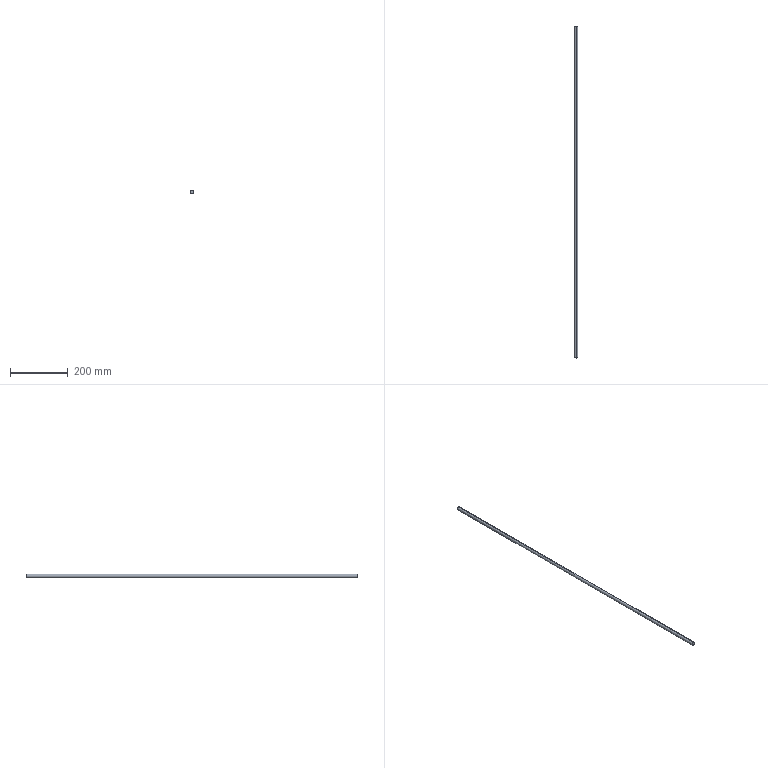Component | SolidWorks | JL001-05-01-002-1 | 1 solid | 4 faces | box 12 x 1150 x 12 mm | volume 130062 mm3 | cylinder 2 | plane 2 | commonest cylinder face diameters 12 x2
build123d program:
from build123d import *

# Parameters (mm, degrees)
SKETCH1_R           = 6
BOSS_EXTRUDE1_DEPTH = 1150


with BuildPart() as part:
    # Sketch1 → Boss-Extrude1 (new body)
    with BuildSketch(Plane(origin=(0, 0, 0), x_dir=(1, 0, 0), z_dir=(0, 1, 0))):
        with Locations(Location((0, 0, 0), (0, 0, 270))):
            Circle(SKETCH1_R)
    extrude(amount=BOSS_EXTRUDE1_DEPTH)


solid = part.part

# Placed as in the assembly
solid = solid.moved(Location((0, -10, 105), (0, 0, 0)))
STEP:
#1=CARTESIAN_POINT('',(0.,44.882,4.37));
#2=VERTEX_POINT('',#1);
#3=CARTESIAN_POINT('',(0.,44.882,3.898));
#4=VERTEX_POINT('',#3);
#5=CARTESIAN_POINT('',(0.,44.882,4.134));
#6=DIRECTION('',(0.,1.,0.));
#7=DIRECTION('',(0.,0.,1.));
#8=AXIS2_PLACEMENT_3D('',#5,#6,#7);
#9=CIRCLE('',#8,0.2362);
#10=EDGE_CURVE('',#2,#4,#9,.T.);
#11=ORIENTED_EDGE('',*,*,#10,.F.);
#12=CARTESIAN_POINT('',(0.,-0.3937,4.37));
#13=VERTEX_POINT('',#12);
#14=CARTESIAN_POINT('',(0.,44.882,4.37));
#15=DIRECTION('',(0.,-1.,0.));
#16=VECTOR('',#15,39.37);
#17=LINE('',#14,#16);
#18=EDGE_CURVE('',#2,#13,#17,.T.);
#19=ORIENTED_EDGE('',*,*,#18,.T.);
#20=CARTESIAN_POINT('',(0.,-0.3937,3.898));
#21=VERTEX_POINT('',#20);
#22=CARTESIAN_POINT('',(0.,-0.3937,4.134));
#23=DIRECTION('',(0.,1.,0.));
#24=DIRECTION('',(0.,0.,1.));
#25=AXIS2_PLACEMENT_3D('',#22,#23,#24);
#26=CIRCLE('',#25,0.2362);
#27=EDGE_CURVE('',#13,#21,#26,.T.);
#28=ORIENTED_EDGE('',*,*,#27,.T.);
#29=CARTESIAN_POINT('',(0.,44.882,3.898));
#30=DIRECTION('',(0.,-1.,0.));
#31=VECTOR('',#30,39.37);
#32=LINE('',#29,#31);
#33=EDGE_CURVE('',#4,#21,#32,.T.);
#34=ORIENTED_EDGE('',*,*,#33,.F.);
#35=EDGE_LOOP('',(#11,#19,#28,#34));
#36=FACE_OUTER_BOUND('',#35,.T.);
#37=CARTESIAN_POINT('',(0.,44.882,4.134));
#38=DIRECTION('',(0.,-1.,0.));
#39=DIRECTION('',(0.,0.,-1.));
#40=AXIS2_PLACEMENT_3D('',#37,#38,#39);
#41=CYLINDRICAL_SURFACE('',#40,0.2362);
#42=ADVANCED_FACE('',(#36),#41,.T.);
#43=ORIENTED_EDGE('',*,*,#18,.F.);
#44=CARTESIAN_POINT('',(0.,44.882,4.134));
#45=DIRECTION('',(0.,1.,0.));
#46=DIRECTION('',(0.,0.,1.));
#47=AXIS2_PLACEMENT_3D('',#44,#45,#46);
#48=CIRCLE('',#47,0.2362);
#49=EDGE_CURVE('',#4,#2,#48,.T.);
#50=ORIENTED_EDGE('',*,*,#49,.F.);
#51=ORIENTED_EDGE('',*,*,#33,.T.);
#52=CARTESIAN_POINT('',(0.,-0.3937,4.134));
#53=DIRECTION('',(0.,1.,0.));
#54=DIRECTION('',(0.,0.,1.));
#55=AXIS2_PLACEMENT_3D('',#52,#53,#54);
#56=CIRCLE('',#55,0.2362);
#57=EDGE_CURVE('',#21,#13,#56,.T.);
#58=ORIENTED_EDGE('',*,*,#57,.T.);
#59=EDGE_LOOP('',(#43,#50,#51,#58));
#60=FACE_OUTER_BOUND('',#59,.T.);
#61=CARTESIAN_POINT('',(0.,44.882,4.134));
#62=DIRECTION('',(0.,-1.,0.));
#63=DIRECTION('',(0.,0.,-1.));
#64=AXIS2_PLACEMENT_3D('',#61,#62,#63);
#65=CYLINDRICAL_SURFACE('',#64,0.2362);
#66=ADVANCED_FACE('',(#60),#65,.T.);
#67=ORIENTED_EDGE('',*,*,#49,.T.);
#68=ORIENTED_EDGE('',*,*,#10,.T.);
#69=EDGE_LOOP('',(#67,#68));
#70=FACE_OUTER_BOUND('',#69,.T.);
#71=CARTESIAN_POINT('',(0.,44.882,4.134));
#72=DIRECTION('',(0.,1.,0.));
#73=DIRECTION('',(0.,0.,1.));
#74=AXIS2_PLACEMENT_3D('',#71,#72,#73);
#75=PLANE('',#74);
#76=ADVANCED_FACE('',(#70),#75,.T.);
#77=ORIENTED_EDGE('',*,*,#57,.F.);
#78=ORIENTED_EDGE('',*,*,#27,.F.);
#79=EDGE_LOOP('',(#77,#78));
#80=FACE_OUTER_BOUND('',#79,.T.);
#81=CARTESIAN_POINT('',(0.,-0.3937,4.134));
#82=DIRECTION('',(0.,1.,0.));
#83=DIRECTION('',(0.,0.,1.));
#84=AXIS2_PLACEMENT_3D('',#81,#82,#83);
#85=PLANE('',#84);
#86=ADVANCED_FACE('',(#80),#85,.F.);
#87=CLOSED_SHELL('',(#42,#66,#76,#86));
#88=MANIFOLD_SOLID_BREP('',#87);
#89=CARTESIAN_POINT('',(0.,0.,0.));
#90=DIRECTION('',(0.,0.,1.));
#91=DIRECTION('',(1.,0.,0.));
#92=AXIS2_PLACEMENT_3D('',#89,#90,#91);
#93=(LENGTH_UNIT()NAMED_UNIT(*)SI_UNIT($,.METRE.));
#94=LENGTH_MEASURE_WITH_UNIT(LENGTH_MEASURE(0.0254),#93);
#95=DIMENSIONAL_EXPONENTS(1.,0.,0.,0.,0.,0.,0.);
#96=(CONVERSION_BASED_UNIT('',#94)LENGTH_UNIT()NAMED_UNIT(#95));
#97=UNCERTAINTY_MEASURE_WITH_UNIT(LENGTH_MEASURE(0.00001),#96,'','');
#98=(NAMED_UNIT(*)PLANE_ANGLE_UNIT()SI_UNIT($,.RADIAN.));
#99=(NAMED_UNIT(*)SI_UNIT($,.STERADIAN.)SOLID_ANGLE_UNIT());
#100=(GEOMETRIC_REPRESENTATION_CONTEXT(3)GLOBAL_UNCERTAINTY_ASSIGNED_CONTEXT((#97))GLOBAL_UNIT_ASSIGNED_CONTEXT((#96,#98,#99))REPRESENTATION_CONTEXT('',''));
#101=ADVANCED_BREP_SHAPE_REPRESENTATION('',(#88,#92),#100);
#102=COLOUR_RGB('',0.7922,0.8196,0.9333);
#103=FILL_AREA_STYLE_COLOUR('',#102);
#104=FILL_AREA_STYLE('',(#103));
#105=SURFACE_STYLE_FILL_AREA(#104);
#106=SURFACE_SIDE_STYLE('',(#105));
#107=SURFACE_STYLE_USAGE(.BOTH.,#106);
#108=PRESENTATION_STYLE_ASSIGNMENT((#107));
#109=STYLED_ITEM('',(#108),#88);
#110=PRESENTATION_LAYER_ASSIGNMENT('','',(#109));
#111=(LENGTH_UNIT()NAMED_UNIT(*)SI_UNIT($,.METRE.));
#112=LENGTH_MEASURE_WITH_UNIT(LENGTH_MEASURE(0.0254),#111);
#113=DIMENSIONAL_EXPONENTS(1.,0.,0.,0.,0.,0.,0.);
#114=(CONVERSION_BASED_UNIT('',#112)LENGTH_UNIT()NAMED_UNIT(#113));
#115=UNCERTAINTY_MEASURE_WITH_UNIT(LENGTH_MEASURE(0.00001),#114,'','');
#116=(NAMED_UNIT(*)PLANE_ANGLE_UNIT()SI_UNIT($,.RADIAN.));
#117=(NAMED_UNIT(*)SI_UNIT($,.STERADIAN.)SOLID_ANGLE_UNIT());
#118=(GEOMETRIC_REPRESENTATION_CONTEXT(3)GLOBAL_UNCERTAINTY_ASSIGNED_CONTEXT((#115))GLOBAL_UNIT_ASSIGNED_CONTEXT((#114,#116,#117))REPRESENTATION_CONTEXT('',''));
#119=MECHANICAL_DESIGN_GEOMETRIC_PRESENTATION_REPRESENTATION('',(#109),#118);